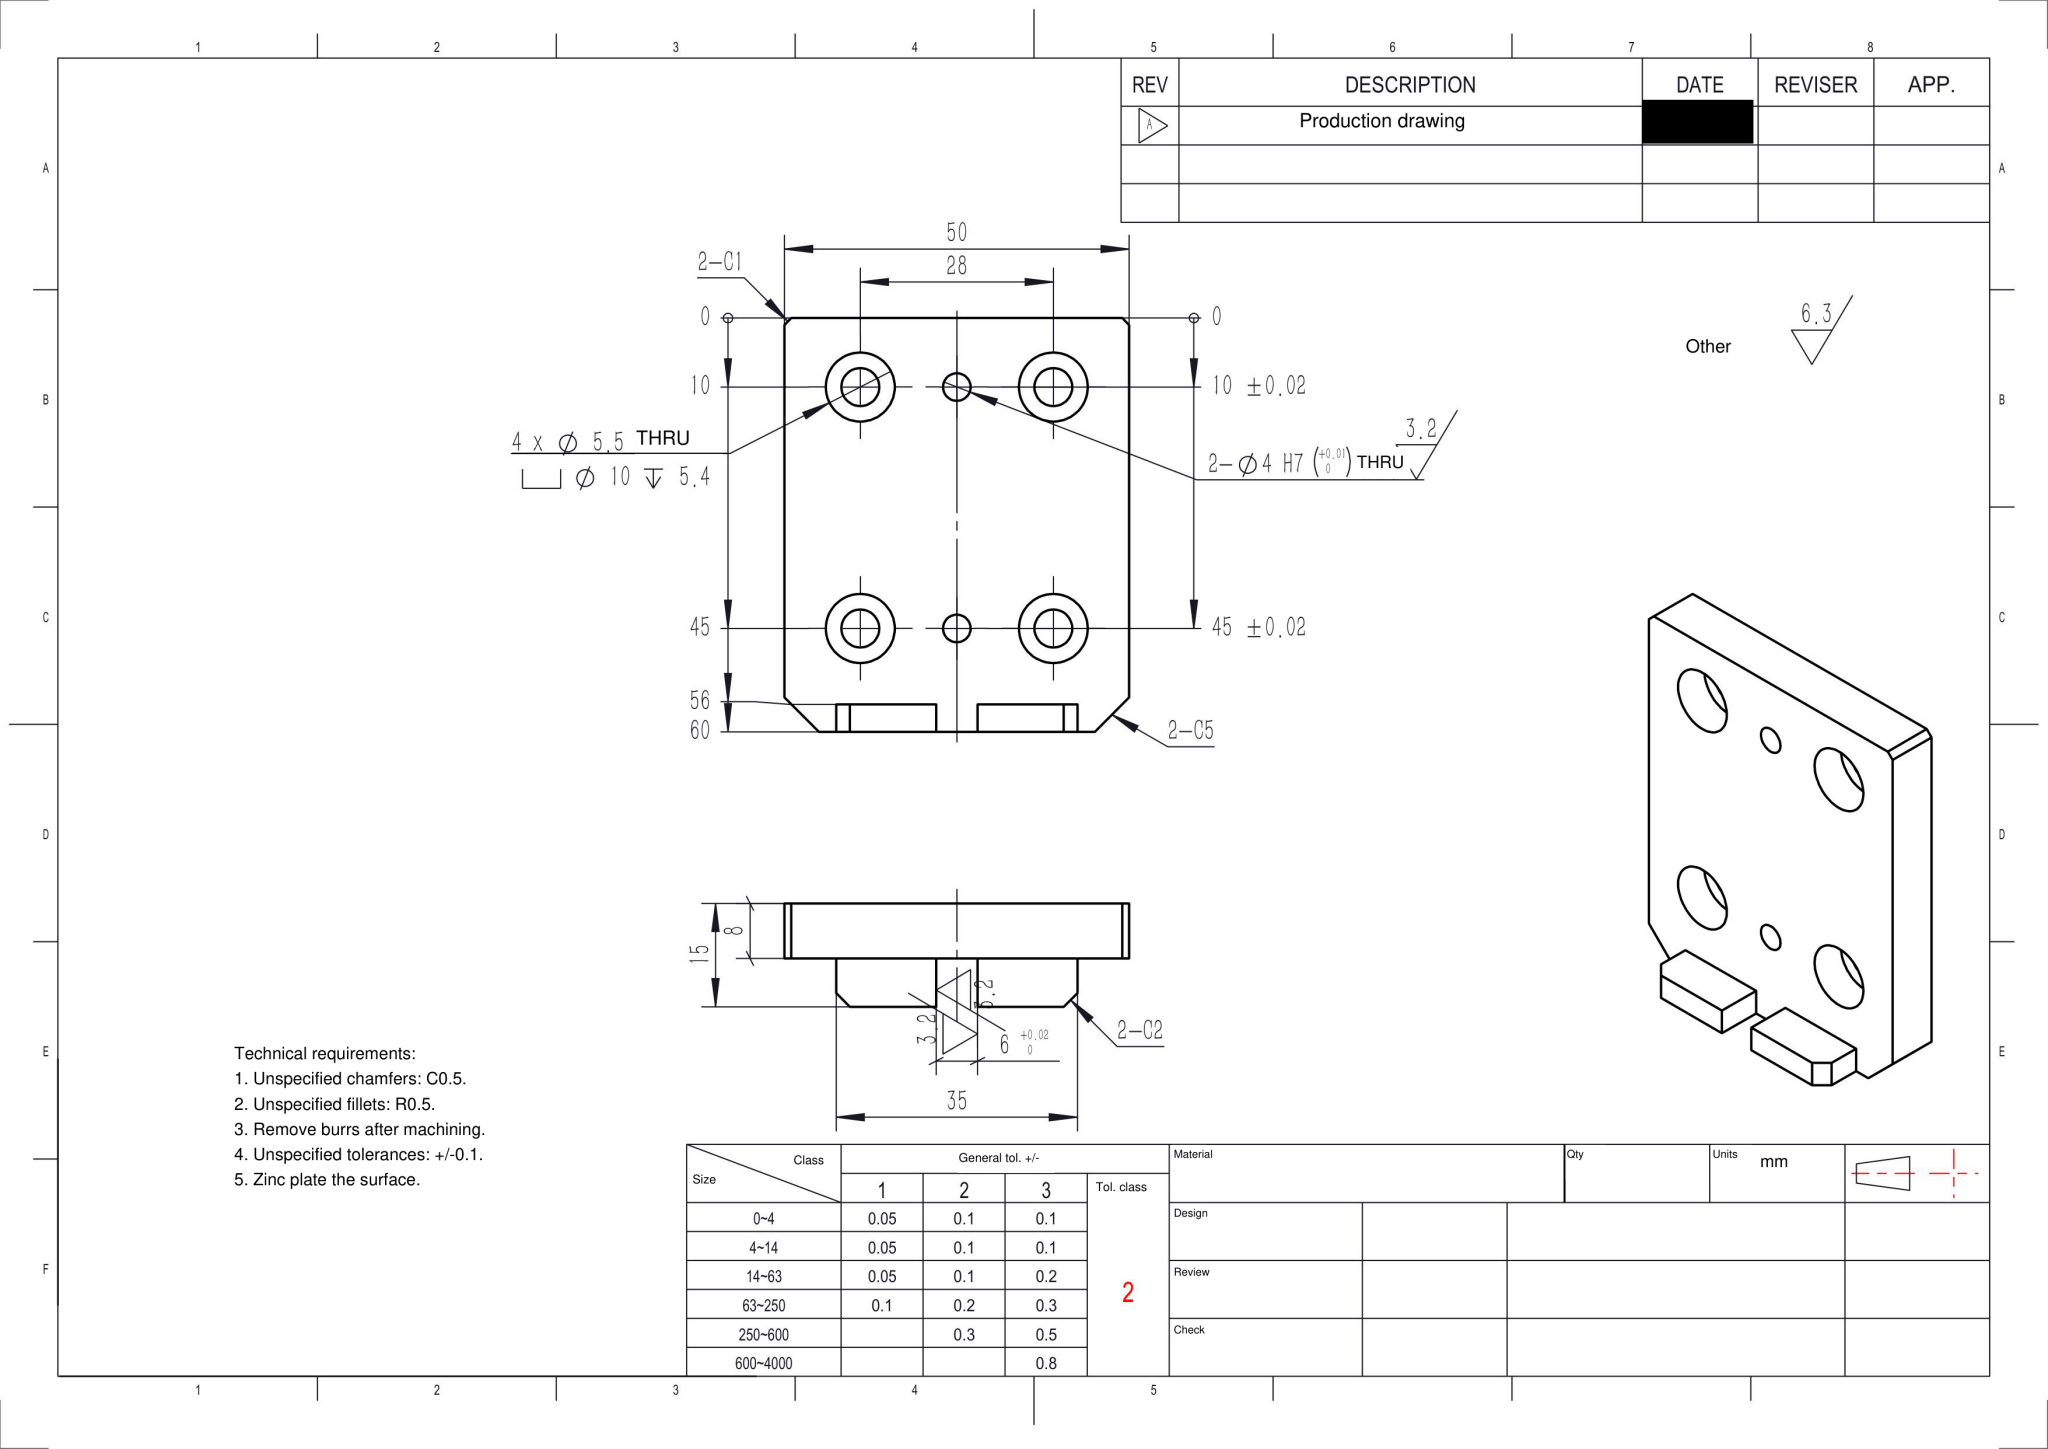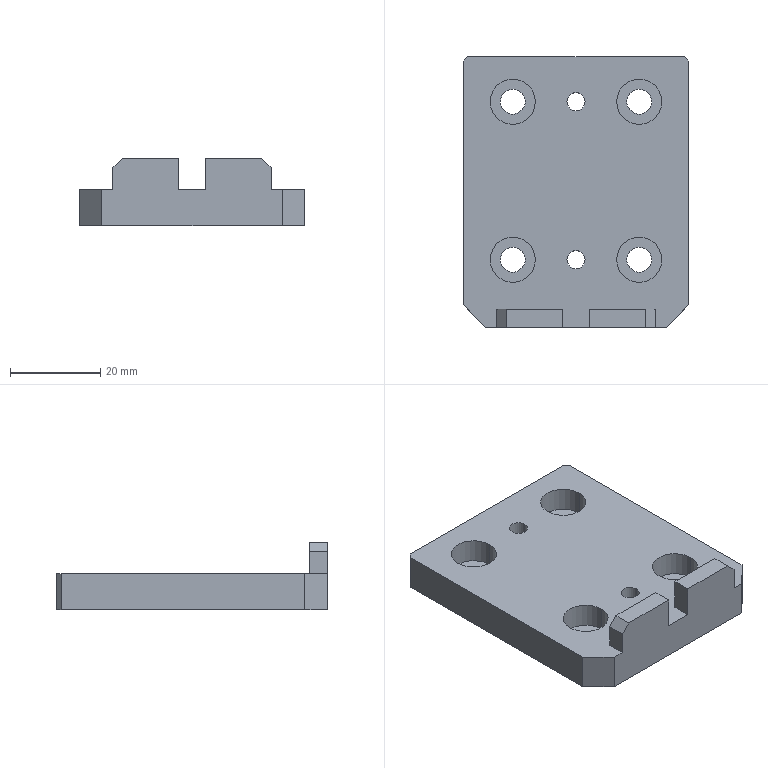Part | NX | mm | 1 solid | 44 faces | box 50 x 60 x 15 mm | volume 22443 mm3 | plane 24 | cylinder 20 | commonest cylinder face diameters 10 x8 5.5 x8 4 x4